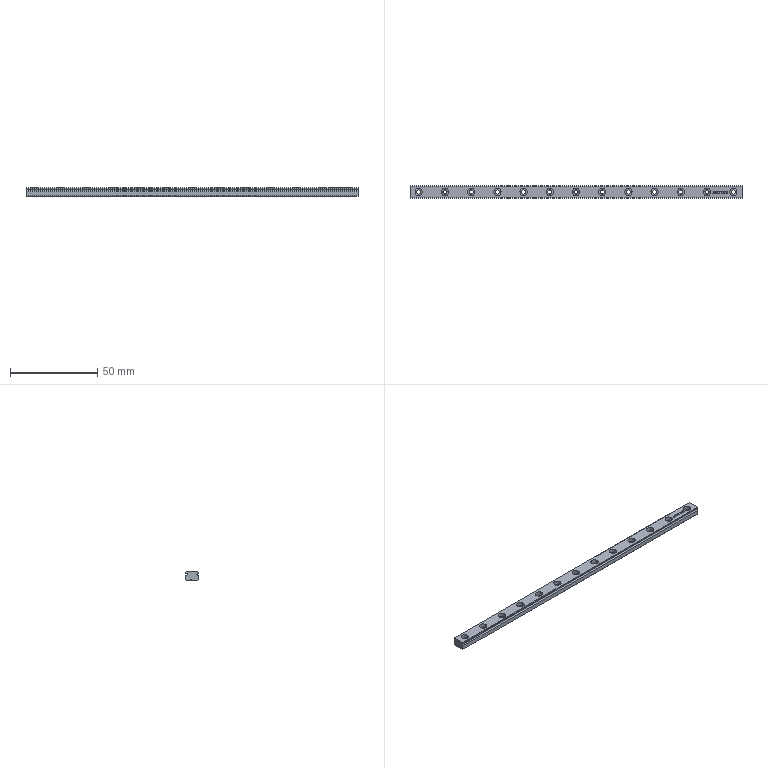Component | SolidWorks | GuideRail-1_LinearGuideMGN7(HIWIN)-1 | 1 solid | 189 faces | box 190 x 7 x 4.8 mm | volume 5492 mm3 | plane 111 | cylinder 69 | spline 9 | commonest cylinder face diameters 4.2 x26 2.4 x26 0.6 x14 1.4 x3 | material Chrome Stainless Steel
build123d program:
from build123d import *

# Parameters (mm, degrees)
BOSS_EXTRUDE1_DEPTH                             = 190
M2_HEX_SOCKET_HEAD_CAP_SCREW_CBORE1_D           = 2.4
M2_HEX_SOCKET_HEAD_CAP_SCREW_CBORE1_CBORE_D     = 4.2
M2_HEX_SOCKET_HEAD_CAP_SCREW_CBORE1_CBORE_DEPTH = 2.3
LPATTERN1_COUNT                                 = 13
LPATTERN1_PITCH                                 = 15
SKETCH6_W                                       = 1
SKETCH6_H                                       = 0.08974
CUT_EXTRUDE1_DEPTH                              = 0.1


with BuildPart() as part:
    # Sketch1 → Boss-Extrude1 (new body)
    with BuildSketch(Plane.XY):
        with BuildLine():
            Line((-3.5, 4.6), (-3.5, 4))
            ThreePointArc((-3.5, 4), (-2.8, 3.3), (-3.5, 2.6))
            Line((-3.5, 2.6), (-3.5, 0.2))
            Line((-3.5, 0.2), (-3.3, 0))
            Line((-3.3, 0), (0.2, 0))
            ThreePointArc((0.2, 0), (0.5, 0.3), (0.8, 0))
            Line((0.8, 0), (3.3, 0))
            Line((3.3, 0), (3.5, 0.2))
            Line((3.5, 0.2), (3.5, 2.6))
            ThreePointArc((3.5, 2.6), (2.8, 3.3), (3.5, 4))
            Line((3.5, 4), (3.5, 4.6))
            Line((3.5, 4.6), (3.3, 4.8))
            Line((3.3, 4.8), (-3.3, 4.8))
            Line((-3.3, 4.8), (-3.5, 4.6))
        make_face()
    extrude(amount=-BOSS_EXTRUDE1_DEPTH)

    # M2 Hex Socket Head Cap Screw CBORE1 (through all)
    with Locations(Plane(origin=(1.648, 4.8, 19.977), x_dir=(-1, 0, 0), z_dir=(0, 1, 0))):
        with Locations((1.648, -24.977)):
            m2_hex_socket_head_cap_screw_cbore1 = CounterBoreHole(M2_HEX_SOCKET_HEAD_CAP_SCREW_CBORE1_D / 2, M2_HEX_SOCKET_HEAD_CAP_SCREW_CBORE1_CBORE_D / 2, M2_HEX_SOCKET_HEAD_CAP_SCREW_CBORE1_CBORE_DEPTH)

    # LPattern1: M2 Hex Socket Head Cap Screw CBORE1 ×13
    with Locations(*[(0, 0, -i * LPATTERN1_PITCH) for i in range(1, LPATTERN1_COUNT)]):
        add(m2_hex_socket_head_cap_screw_cbore1, mode=Mode.SUBTRACT)

    # Sketch6 → Cut-Extrude1 (cut)
    with BuildSketch(Plane(origin=(0, 4.8, 0), x_dir=(1, 0, 0), z_dir=(0, 1, 0))):
        Polygon((-1, 8.327), (-1, 8.417), (-0.5897, 8.417), (-0.5897, 8.929), (-1, 8.929), (-1, 9.019), (0, 9.019), (0, 8.929), (-0.4872, 8.929), (-0.4872, 8.417), (0, 8.417), (0, 8.327), align=None)
        with Locations((-0.5, 9.321)):
            Rectangle(SKETCH6_W, SKETCH6_H)
        Polygon((-1, 9.519), (-1, 9.612), (-0.2666, 9.808), (-1, 10.099), (-1, 10.112), (-0.2716, 10.397), (-1, 10.594), (-1, 10.686), (0, 10.416), (0, 10.403), (-0.7648, 10.103), (0, 9.798), (0, 9.785), align=None)
        with Locations((-0.5, 10.962)):
            Rectangle(SKETCH6_W, SKETCH6_H)
        Polygon((0, 11.224), (-1, 11.224), (-1, 11.243), (-0.2129, 11.904), (-1, 11.904), (-1, 11.994), (0, 11.994), (0, 11.973), (-0.7853, 11.314), (0, 11.314), align=None)
        Polygon((0, 12.583), (-1, 12.715), (-1, 12.728), (-0.1795, 13.141), (-1, 13.553), (-1, 13.566), (0, 13.699), (0, 13.609), (-0.7196, 13.513), (0, 13.152), (0, 13.132), (-0.7212, 12.769), (0, 12.674), align=None)
        with BuildLine():
            Line((-0.8293, 14.84), (-0.7564, 14.763))
            add(Edge.make_bspline(
                [(-0.7564, 14.763), (-0.7695, 14.749), (-0.7954, 14.721), (-0.8289, 14.676), (-0.8579, 14.63), (-0.8814, 14.581), (-0.8997, 14.532), (-0.9131, 14.483), (-0.9216, 14.435), (-0.9226, 14.403), (-0.9231, 14.387)],
                knots=[0, 0, 0, 0, 1.089, 2.152, 3.19, 4.218, 5.218, 6.174, 7.1, 8, 8, 8, 8], degree=3))
            add(Edge.make_bspline(
                [(-0.9231, 14.387), (-0.923, 14.378), (-0.9227, 14.358), (-0.9197, 14.33), (-0.9154, 14.301), (-0.9091, 14.273), (-0.9012, 14.245), (-0.8912, 14.218), (-0.8796, 14.191), (-0.8662, 14.164), (-0.8515, 14.139), (-0.8352, 14.115), (-0.8179, 14.092), (-0.799, 14.07), (-0.7788, 14.051), (-0.7576, 14.032), (-0.7351, 14.015), (-0.7113, 14), (-0.6868, 13.987), (-0.6617, 13.975), (-0.6364, 13.965), (-0.6106, 13.957), (-0.5845, 13.95), (-0.5582, 13.946), (-0.5314, 13.943), (-0.5134, 13.943), (-0.5044, 13.942)],
                knots=[0, 0, 0, 0, 1.028, 2.054, 3.065, 4.081, 5.107, 6.131, 7.173, 8.228, 9.276, 10.308, 11.325, 12.329, 13.321, 14.316, 15.309, 16.309, 17.306, 18.285, 19.246, 20.203, 21.146, 22.095, 23.042, 24, 24, 24, 24], degree=3))
            add(Edge.make_bspline(
                [(-0.5044, 13.942), (-0.4952, 13.943), (-0.4768, 13.943), (-0.4493, 13.946), (-0.4222, 13.951), (-0.3955, 13.958), (-0.3691, 13.966), (-0.3431, 13.977), (-0.3174, 13.99), (-0.2923, 14.004), (-0.2678, 14.02), (-0.2446, 14.038), (-0.2229, 14.058), (-0.2024, 14.078), (-0.1832, 14.1), (-0.1655, 14.124), (-0.1491, 14.149), (-0.1341, 14.176), (-0.1207, 14.204), (-0.1088, 14.232), (-0.09905, 14.261), (-0.09107, 14.291), (-0.08452, 14.321), (-0.08031, 14.352), (-0.07726, 14.384), (-0.07704, 14.406), (-0.07692, 14.416)],
                knots=[0, 0, 0, 0, 0.9359, 1.869, 2.8, 3.73, 4.665, 5.616, 6.583, 7.57, 8.563, 9.553, 10.533, 11.515, 12.51, 13.508, 14.526, 15.561, 16.601, 17.643, 18.681, 19.72, 20.772, 21.833, 22.908, 24, 24, 24, 24], degree=3))
            add(Edge.make_bspline(
                [(-0.07692, 14.416), (-0.07719, 14.429), (-0.07773, 14.455), (-0.08187, 14.492), (-0.08834, 14.528), (-0.09783, 14.562), (-0.1099, 14.595), (-0.1247, 14.627), (-0.1423, 14.656), (-0.1622, 14.685), (-0.1843, 14.71), (-0.208, 14.734), (-0.2336, 14.754), (-0.2606, 14.772), (-0.2893, 14.787), (-0.3196, 14.799), (-0.3515, 14.808), (-0.3735, 14.812), (-0.3846, 14.814)],
                knots=[0, 0, 0, 0, 1.13, 2.219, 3.279, 4.312, 5.323, 6.328, 7.327, 8.334, 9.329, 10.292, 11.241, 12.174, 13.112, 14.052, 15.016, 16, 16, 16, 16], degree=3))
            Line((-0.3846, 14.814), (-0.3846, 14.481))
            Line((-0.3846, 14.481), (-0.4872, 14.481))
            Line((-0.4872, 14.481), (-0.4872, 14.904))
            add(Edge.make_bspline(
                [(-0.4872, 14.904), (-0.4681, 14.903), (-0.4306, 14.902), (-0.3761, 14.896), (-0.3246, 14.885), (-0.276, 14.87), (-0.2305, 14.851), (-0.188, 14.828), (-0.1487, 14.8), (-0.1124, 14.769), (-0.08002, 14.734), (-0.05156, 14.696), (-0.02759, 14.655), (-0.008086, 14.611), (0.007135, 14.564), (0.01793, 14.515), (0.02439, 14.463), (0.02522, 14.427), (0.02564, 14.408)],
                knots=[0, 0, 0, 0, 1.14, 2.232, 3.274, 4.278, 5.255, 6.214, 7.164, 8.118, 9.068, 10.008, 10.945, 11.892, 12.865, 13.864, 14.908, 16, 16, 16, 16], degree=3))
            add(Edge.make_bspline(
                [(0.02564, 14.408), (0.02548, 14.397), (0.02516, 14.375), (0.02288, 14.342), (0.01937, 14.31), (0.01407, 14.279), (0.007581, 14.249), (-0.0007293, 14.219), (-0.01035, 14.191), (-0.02129, 14.163), (-0.03397, 14.137), (-0.04806, 14.111), (-0.06348, 14.086), (-0.08051, 14.062), (-0.09902, 14.039), (-0.119, 14.017), (-0.1405, 13.995), (-0.1558, 13.982), (-0.1635, 13.975)],
                knots=[0, 0, 0, 0, 1.108, 2.185, 3.234, 4.263, 5.276, 6.27, 7.252, 8.226, 9.19, 10.146, 11.103, 12.066, 13.032, 14.011, 14.998, 16, 16, 16, 16], degree=3))
            add(Edge.make_bspline(
                [(-0.1635, 13.975), (-0.1757, 13.965), (-0.1998, 13.946), (-0.2386, 13.921), (-0.2787, 13.9), (-0.3203, 13.883), (-0.3633, 13.869), (-0.4078, 13.859), (-0.4536, 13.854), (-0.4847, 13.853), (-0.5004, 13.853)],
                knots=[0, 0, 0, 0, 1.023, 2.029, 3.014, 3.995, 4.976, 5.966, 6.971, 8, 8, 8, 8], degree=3))
            add(Edge.make_bspline(
                [(-0.5004, 13.853), (-0.5122, 13.853), (-0.5355, 13.853), (-0.5702, 13.857), (-0.6043, 13.862), (-0.6378, 13.87), (-0.6706, 13.879), (-0.7028, 13.892), (-0.7344, 13.906), (-0.7652, 13.922), (-0.7949, 13.94), (-0.8231, 13.96), (-0.8496, 13.982), (-0.8743, 14.005), (-0.8976, 14.03), (-0.919, 14.057), (-0.9389, 14.085), (-0.9569, 14.115), (-0.9731, 14.145), (-0.9872, 14.177), (-0.9989, 14.211), (-1.009, 14.245), (-1.016, 14.28), (-1.022, 14.316), (-1.025, 14.353), (-1.025, 14.378), (-1.026, 14.39)],
                knots=[0, 0, 0, 0, 1.009, 2.005, 2.991, 3.967, 4.948, 5.927, 6.92, 7.92, 8.923, 9.906, 10.883, 11.852, 12.825, 13.799, 14.781, 15.774, 16.776, 17.772, 18.776, 19.79, 20.809, 21.852, 22.911, 24, 24, 24, 24], degree=3))
            add(Edge.make_bspline(
                [(-1.026, 14.39), (-1.025, 14.401), (-1.025, 14.421), (-1.023, 14.452), (-1.019, 14.482), (-1.014, 14.512), (-1.008, 14.541), (-0.9996, 14.569), (-0.9903, 14.598), (-0.9791, 14.625), (-0.9665, 14.653), (-0.9523, 14.68), (-0.9362, 14.707), (-0.9183, 14.734), (-0.8987, 14.761), (-0.8771, 14.787), (-0.8542, 14.814), (-0.8377, 14.831), (-0.8293, 14.84)],
                knots=[0, 0, 0, 0, 0.9859, 1.955, 2.915, 3.87, 4.815, 5.76, 6.705, 7.649, 8.608, 9.583, 10.581, 11.604, 12.66, 13.74, 14.853, 16, 16, 16, 16], degree=3))
        make_face()
        Polygon((0, 15.109), (-1, 15.109), (-1, 15.128), (-0.2129, 15.788), (-1, 15.788), (-1, 15.878), (0, 15.878), (0, 15.858), (-0.7853, 15.199), (0, 15.199), align=None)
        Polygon((-1, 16.109), (-1, 16.724), (0.02564, 16.199), (-0.01703, 16.121), (-0.8974, 16.573), (-0.8974, 16.109), align=None)
    extrude(amount=-CUT_EXTRUDE1_DEPTH, mode=Mode.SUBTRACT)


solid = part.part

# Placed as in the assembly
solid = solid.moved(Location((91.222, 32.633, 83), (90, 90, 0)))